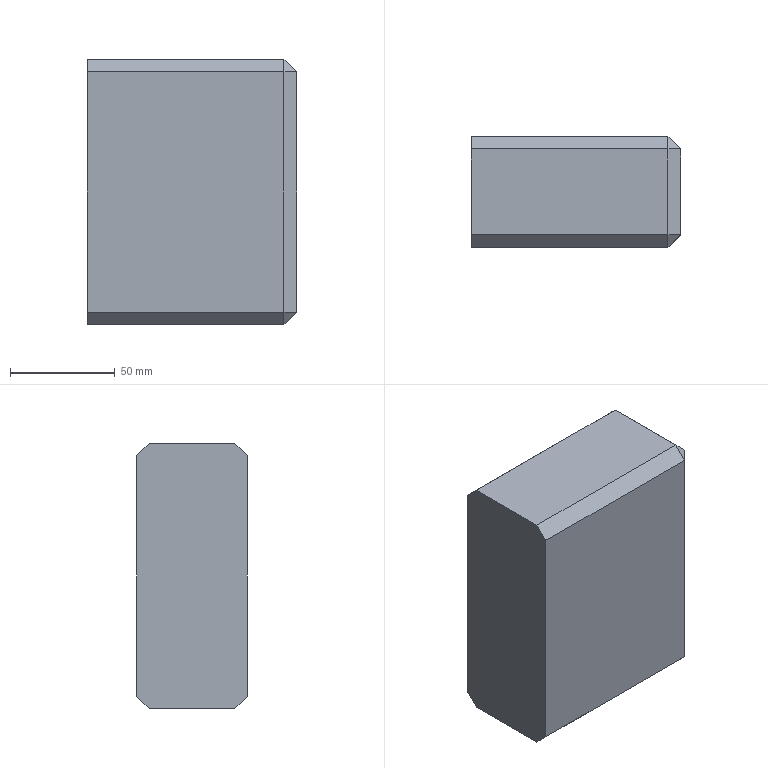Component | NX | MOTOR_BOX | 1 solid | 36 faces | volume 45722 mm3 | plane 36